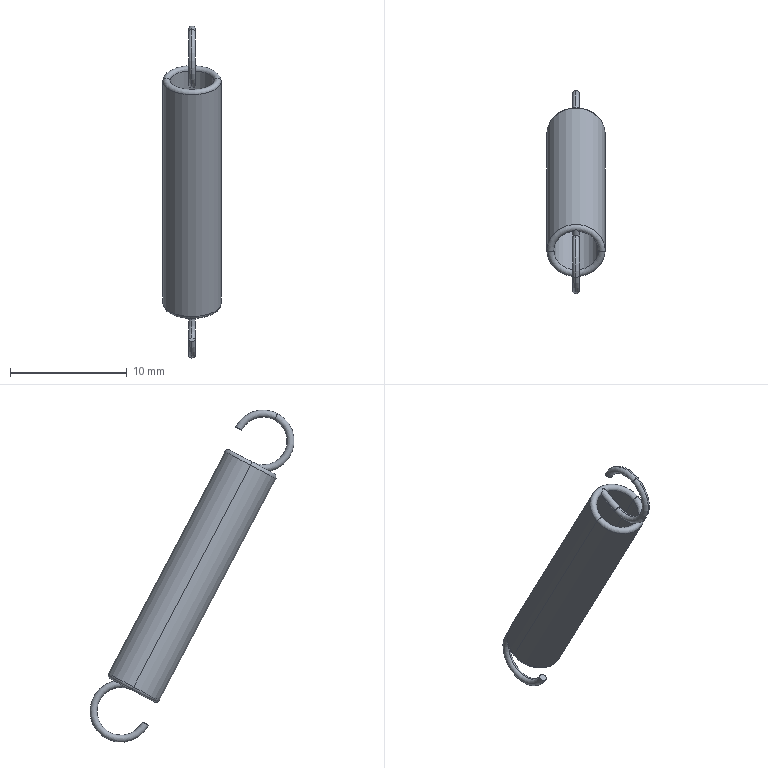Component | SolidWorks | LiftingPlateAssembly-1_AWS5_30-2 | 1 solid | 20 faces | box 5 x 17.5 x 28.48 mm | volume 190 mm3 | torus 10 | cylinder 8 | plane 2 | commonest cylinder face diameters 0.6 x4 5 x2 3.8 x2
build123d program:
from build123d import *

# Parameters (mm, degrees)
SKETCH2_W      = 0.3
SKETCH2_H      = 2.2
SKETCH3_R      = 0.3
REVOLVE3_ANGLE = 271
SKETCH4_W      = 0.3
SKETCH4_H      = 2.2
SKETCH5_R      = 0.3
REVOLVE5_ANGLE = 271


with BuildPart() as part:
    # Sketch1 → Revolve1 (revolve)
    with BuildSketch(Plane.XY, mode=Mode.PRIVATE) as revolve1_sk:
        with BuildLine():
            Line((4.25, 2.5), (25.75, 2.5))
            ThreePointArc((25.75, 2.5), (26.05, 2.2), (25.75, 1.9))
            Line((25.75, 1.9), (4.25, 1.9))
            ThreePointArc((4.25, 1.9), (3.95, 2.2), (4.25, 2.5))
        make_face()
    revolve(revolve1_sk.sketch.rotate(Axis((26.2, 0, 0), (-1, 0, 0)), 270), axis=Axis((26.2, 0, 0), (-1, 0, 0)))

    # Sketch2 → Revolve2 (revolve)
    with BuildSketch(Plane.XY, mode=Mode.PRIVATE) as revolve2_sk:
        with Locations((25.9, 1.1)):
            Rectangle(SKETCH2_W, SKETCH2_H)
    revolve(revolve2_sk.sketch.rotate(Axis((25.75, 0, 0), (0, 1, 0)), 270), axis=Axis((25.75, 0, 0), (0, 1, 0)))

    # Sketch3 → Revolve3 (revolve)
    with BuildSketch(Plane(origin=(0, 0, 0), x_dir=(1, 0, 0), z_dir=(0, 1, 0))):
        with Locations(Location((25.75, 0, 0), (0, 0, 270))):
            Circle(SKETCH3_R)
    revolve(axis=Axis((28.1, 0, -2.5), (0, 0, 1)), revolution_arc=REVOLVE3_ANGLE)

    # Sketch4 → Revolve4 (revolve)
    with BuildSketch(Plane.XY, mode=Mode.PRIVATE) as revolve4_sk:
        with Locations((4.4, -1.1)):
            Rectangle(SKETCH4_W, SKETCH4_H)
    revolve(revolve4_sk.sketch.rotate(Axis((4.25, 0, 0), (0, -1, 0)), 90), axis=Axis((4.25, 0, 0), (0, -1, 0)))

    # Sketch5 → Revolve5 (revolve)
    with BuildSketch(Plane(origin=(0, 0, 0), x_dir=(1, 0, 0), z_dir=(0, 1, 0))):
        with Locations(Location((4.25, 0, 0), (0, 0, 270))):
            Circle(SKETCH5_R)
    revolve(axis=Axis((1.9, 0, 2.5), (0, 0, 1)), revolution_arc=REVOLVE5_ANGLE)


solid = part.part

# Placed as in the assembly
solid = solid.moved(Location((-282.5, -21.911, -69.866), (27.761, -90, 0)))
STEP:
#1=CARTESIAN_POINT('',(-11.122,-1.427,-1.679));
#2=VERTEX_POINT('',#1);
#3=CARTESIAN_POINT('',(-11.122,-1.416,-1.7));
#4=VERTEX_POINT('',#3);
#5=CARTESIAN_POINT('',(-11.122,-1.421,-1.69));
#6=DIRECTION('',(-0.,0.8849,0.4658));
#7=DIRECTION('',(0.,-0.4658,0.8849));
#8=AXIS2_PLACEMENT_3D('',#5,#6,#7);
#9=CIRCLE('',#8,0.01181);
#10=EDGE_CURVE('',#2,#4,#9,.T.);
#11=ORIENTED_EDGE('',*,*,#10,.F.);
#12=CARTESIAN_POINT('',(-11.122,-1.329,-1.864));
#13=VERTEX_POINT('',#12);
#14=CARTESIAN_POINT('',(-11.122,-1.378,-1.772));
#15=DIRECTION('',(1.,0.,-0.));
#16=DIRECTION('',(0.,1.,0.));
#17=AXIS2_PLACEMENT_3D('',#14,#15,#16);
#18=CIRCLE('',#17,0.1043);
#19=EDGE_CURVE('',#2,#13,#18,.T.);
#20=ORIENTED_EDGE('',*,*,#19,.T.);
#21=CARTESIAN_POINT('',(-11.11,-1.335,-1.854));
#22=VERTEX_POINT('',#21);
#23=CARTESIAN_POINT('',(-11.122,-1.335,-1.854));
#24=DIRECTION('',(0.,-0.8849,-0.4658));
#25=DIRECTION('',(-1.,0.,0.));
#26=AXIS2_PLACEMENT_3D('',#23,#24,#25);
#27=CIRCLE('',#26,0.01181);
#28=EDGE_CURVE('',#13,#22,#27,.T.);
#29=ORIENTED_EDGE('',*,*,#28,.T.);
#30=CARTESIAN_POINT('',(-11.122,-1.34,-1.843));
#31=VERTEX_POINT('',#30);
#32=CARTESIAN_POINT('',(-11.122,-1.335,-1.854));
#33=DIRECTION('',(0.,-0.8849,-0.4658));
#34=DIRECTION('',(-1.,0.,0.));
#35=AXIS2_PLACEMENT_3D('',#32,#33,#34);
#36=CIRCLE('',#35,0.01181);
#37=EDGE_CURVE('',#22,#31,#36,.T.);
#38=ORIENTED_EDGE('',*,*,#37,.T.);
#39=CARTESIAN_POINT('',(-11.122,-1.378,-1.772));
#40=DIRECTION('',(1.,0.,-0.));
#41=DIRECTION('',(0.,1.,0.));
#42=AXIS2_PLACEMENT_3D('',#39,#40,#41);
#43=CIRCLE('',#42,0.08071);
#44=EDGE_CURVE('',#4,#31,#43,.T.);
#45=ORIENTED_EDGE('',*,*,#44,.F.);
#46=EDGE_LOOP('',(#11,#20,#29,#38,#45));
#47=FACE_OUTER_BOUND('',#46,.T.);
#48=CARTESIAN_POINT('',(-11.122,-1.378,-1.772));
#49=DIRECTION('',(1.,0.,-0.));
#50=DIRECTION('',(0.,-0.4658,0.8849));
#51=AXIS2_PLACEMENT_3D('',#48,#49,#50);
#52=TOROIDAL_SURFACE('',#51,0.09252,0.01181);
#53=ADVANCED_FACE('',(#47),#52,.T.);
#54=CARTESIAN_POINT('',(-11.122,-0.9696,-2.721));
#55=VERTEX_POINT('',#54);
#56=CARTESIAN_POINT('',(-11.122,-0.9907,-2.731));
#57=VERTEX_POINT('',#56);
#58=CARTESIAN_POINT('',(-11.122,-0.9801,-2.726));
#59=DIRECTION('',(-0.,0.4503,-0.8929));
#60=DIRECTION('',(-1.,0.,0.));
#61=AXIS2_PLACEMENT_3D('',#58,#59,#60);
#62=CIRCLE('',#61,0.01181);
#63=EDGE_CURVE('',#55,#57,#62,.T.);
#64=ORIENTED_EDGE('',*,*,#63,.T.);
#65=CARTESIAN_POINT('',(-11.122,-0.9461,-2.592));
#66=VERTEX_POINT('',#65);
#67=CARTESIAN_POINT('',(-11.122,-0.8975,-2.684));
#68=DIRECTION('',(1.,0.,-0.));
#69=DIRECTION('',(0.,1.,0.));
#70=AXIS2_PLACEMENT_3D('',#67,#68,#69);
#71=CIRCLE('',#70,0.1043);
#72=EDGE_CURVE('',#57,#66,#71,.T.);
#73=ORIENTED_EDGE('',*,*,#72,.T.);
#74=CARTESIAN_POINT('',(-11.11,-0.9406,-2.603));
#75=VERTEX_POINT('',#74);
#76=CARTESIAN_POINT('',(-11.122,-0.9406,-2.603));
#77=DIRECTION('',(0.,-0.8849,-0.4658));
#78=DIRECTION('',(-1.,0.,0.));
#79=AXIS2_PLACEMENT_3D('',#76,#77,#78);
#80=CIRCLE('',#79,0.01181);
#81=EDGE_CURVE('',#75,#66,#80,.T.);
#82=ORIENTED_EDGE('',*,*,#81,.F.);
#83=CARTESIAN_POINT('',(-11.122,-0.9351,-2.613));
#84=VERTEX_POINT('',#83);
#85=CARTESIAN_POINT('',(-11.122,-0.9406,-2.603));
#86=DIRECTION('',(0.,-0.8849,-0.4658));
#87=DIRECTION('',(-1.,0.,0.));
#88=AXIS2_PLACEMENT_3D('',#85,#86,#87);
#89=CIRCLE('',#88,0.01181);
#90=EDGE_CURVE('',#84,#75,#89,.T.);
#91=ORIENTED_EDGE('',*,*,#90,.F.);
#92=CARTESIAN_POINT('',(-11.122,-0.8975,-2.684));
#93=DIRECTION('',(1.,0.,-0.));
#94=DIRECTION('',(0.,1.,0.));
#95=AXIS2_PLACEMENT_3D('',#92,#93,#94);
#96=CIRCLE('',#95,0.08071);
#97=EDGE_CURVE('',#55,#84,#96,.T.);
#98=ORIENTED_EDGE('',*,*,#97,.F.);
#99=EDGE_LOOP('',(#64,#73,#82,#91,#98));
#100=FACE_OUTER_BOUND('',#99,.T.);
#101=CARTESIAN_POINT('',(-11.122,-0.8975,-2.684));
#102=DIRECTION('',(1.,0.,-0.));
#103=DIRECTION('',(0.,-0.4658,0.8849));
#104=AXIS2_PLACEMENT_3D('',#101,#102,#103);
#105=TOROIDAL_SURFACE('',#104,0.09252,0.01181);
#106=ADVANCED_FACE('',(#100),#105,.T.);
#107=CARTESIAN_POINT('',(-11.122,-1.285,-1.725));
#108=VERTEX_POINT('',#107);
#109=CARTESIAN_POINT('',(-11.122,-1.306,-1.735));
#110=VERTEX_POINT('',#109);
#111=CARTESIAN_POINT('',(-11.122,-1.295,-1.73));
#112=DIRECTION('',(-0.,0.4503,-0.8929));
#113=DIRECTION('',(-1.,0.,0.));
#114=AXIS2_PLACEMENT_3D('',#111,#112,#113);
#115=CIRCLE('',#114,0.01181);
#116=EDGE_CURVE('',#108,#110,#115,.T.);
#117=ORIENTED_EDGE('',*,*,#116,.F.);
#118=CARTESIAN_POINT('',(-11.122,-1.378,-1.772));
#119=DIRECTION('',(1.,0.,-0.));
#120=DIRECTION('',(0.,1.,0.));
#121=AXIS2_PLACEMENT_3D('',#118,#119,#120);
#122=CIRCLE('',#121,0.1043);
#123=EDGE_CURVE('',#108,#2,#122,.T.);
#124=ORIENTED_EDGE('',*,*,#123,.T.);
#125=ORIENTED_EDGE('',*,*,#10,.T.);
#126=CARTESIAN_POINT('',(-11.122,-1.378,-1.772));
#127=DIRECTION('',(1.,0.,-0.));
#128=DIRECTION('',(0.,1.,0.));
#129=AXIS2_PLACEMENT_3D('',#126,#127,#128);
#130=CIRCLE('',#129,0.08071);
#131=EDGE_CURVE('',#110,#4,#130,.T.);
#132=ORIENTED_EDGE('',*,*,#131,.F.);
#133=EDGE_LOOP('',(#117,#124,#125,#132));
#134=FACE_OUTER_BOUND('',#133,.T.);
#135=CARTESIAN_POINT('',(-11.122,-1.378,-1.772));
#136=DIRECTION('',(1.,0.,-0.));
#137=DIRECTION('',(0.,-0.4658,0.8849));
#138=AXIS2_PLACEMENT_3D('',#135,#136,#137);
#139=TOROIDAL_SURFACE('',#138,0.09252,0.01181);
#140=ADVANCED_FACE('',(#134),#139,.T.);
#141=ORIENTED_EDGE('',*,*,#123,.F.);
#142=CARTESIAN_POINT('',(-11.122,-1.295,-1.73));
#143=DIRECTION('',(-0.,0.4503,-0.8929));
#144=DIRECTION('',(-1.,0.,0.));
#145=AXIS2_PLACEMENT_3D('',#142,#143,#144);
#146=CIRCLE('',#145,0.01181);
#147=EDGE_CURVE('',#110,#108,#146,.T.);
#148=ORIENTED_EDGE('',*,*,#147,.F.);
#149=ORIENTED_EDGE('',*,*,#131,.T.);
#150=CARTESIAN_POINT('',(-11.122,-1.421,-1.69));
#151=DIRECTION('',(-0.,0.8849,0.4658));
#152=DIRECTION('',(0.,-0.4658,0.8849));
#153=AXIS2_PLACEMENT_3D('',#150,#151,#152);
#154=CIRCLE('',#153,0.01181);
#155=EDGE_CURVE('',#4,#2,#154,.T.);
#156=ORIENTED_EDGE('',*,*,#155,.T.);
#157=EDGE_LOOP('',(#141,#148,#149,#156));
#158=FACE_OUTER_BOUND('',#157,.T.);
#159=CARTESIAN_POINT('',(-11.122,-1.378,-1.772));
#160=DIRECTION('',(1.,0.,-0.));
#161=DIRECTION('',(0.,-0.4658,0.8849));
#162=AXIS2_PLACEMENT_3D('',#159,#160,#161);
#163=TOROIDAL_SURFACE('',#162,0.09252,0.01181);
#164=ADVANCED_FACE('',(#158),#163,.T.);
#165=CARTESIAN_POINT('',(-11.134,-1.269,-1.819));
#166=VERTEX_POINT('',#165);
#167=CARTESIAN_POINT('',(-11.11,-1.269,-1.819));
#168=VERTEX_POINT('',#167);
#169=CARTESIAN_POINT('',(-11.134,-1.269,-1.819));
#170=CARTESIAN_POINT('',(-11.134,-1.268,-1.822));
#171=CARTESIAN_POINT('',(-11.133,-1.266,-1.824));
#172=CARTESIAN_POINT('',(-11.128,-1.264,-1.828));
#173=CARTESIAN_POINT('',(-11.125,-1.263,-1.829));
#174=CARTESIAN_POINT('',(-11.119,-1.263,-1.829));
#175=CARTESIAN_POINT('',(-11.116,-1.264,-1.828));
#176=CARTESIAN_POINT('',(-11.111,-1.266,-1.824));
#177=CARTESIAN_POINT('',(-11.11,-1.268,-1.822));
#178=CARTESIAN_POINT('',(-11.11,-1.269,-1.819));
#179=B_SPLINE_CURVE_WITH_KNOTS('',3,(#169,#170,#171,#172,#173,#174,#175,#176,#177,#178),.UNSPECIFIED.,.F.,.F.,(4,2,2,2,4),(0.,0.0002349,0.0004697,0.0007046,0.0009394),.UNSPECIFIED.);
#180=EDGE_CURVE('',#166,#168,#179,.T.);
#181=ORIENTED_EDGE('',*,*,#180,.T.);
#182=CARTESIAN_POINT('',(-11.11,-1.335,-1.854));
#183=DIRECTION('',(0.,-0.8849,-0.4658));
#184=VECTOR('',#183,39.37);
#185=LINE('',#182,#184);
#186=EDGE_CURVE('',#168,#22,#185,.T.);
#187=ORIENTED_EDGE('',*,*,#186,.T.);
#188=ORIENTED_EDGE('',*,*,#28,.F.);
#189=CARTESIAN_POINT('',(-11.134,-1.335,-1.854));
#190=VERTEX_POINT('',#189);
#191=CARTESIAN_POINT('',(-11.122,-1.335,-1.854));
#192=DIRECTION('',(0.,-0.8849,-0.4658));
#193=DIRECTION('',(-1.,0.,0.));
#194=AXIS2_PLACEMENT_3D('',#191,#192,#193);
#195=CIRCLE('',#194,0.01181);
#196=EDGE_CURVE('',#190,#13,#195,.T.);
#197=ORIENTED_EDGE('',*,*,#196,.F.);
#198=CARTESIAN_POINT('',(-11.134,-1.335,-1.854));
#199=DIRECTION('',(0.,-0.8849,-0.4658));
#200=VECTOR('',#199,39.37);
#201=LINE('',#198,#200);
#202=EDGE_CURVE('',#166,#190,#201,.T.);
#203=ORIENTED_EDGE('',*,*,#202,.F.);
#204=EDGE_LOOP('',(#181,#187,#188,#197,#203));
#205=FACE_OUTER_BOUND('',#204,.T.);
#206=CARTESIAN_POINT('',(-11.122,-1.335,-1.854));
#207=DIRECTION('',(0.,-0.8849,-0.4658));
#208=DIRECTION('',(-1.,0.,0.));
#209=AXIS2_PLACEMENT_3D('',#206,#207,#208);
#210=CYLINDRICAL_SURFACE('',#209,0.01181);
#211=ADVANCED_FACE('',(#205),#210,.T.);
#212=CARTESIAN_POINT('',(-11.134,-0.9406,-2.603));
#213=VERTEX_POINT('',#212);
#214=CARTESIAN_POINT('',(-11.122,-0.9406,-2.603));
#215=DIRECTION('',(0.,-0.8849,-0.4658));
#216=DIRECTION('',(-1.,0.,0.));
#217=AXIS2_PLACEMENT_3D('',#214,#215,#216);
#218=CIRCLE('',#217,0.01181);
#219=EDGE_CURVE('',#213,#84,#218,.T.);
#220=ORIENTED_EDGE('',*,*,#219,.T.);
#221=ORIENTED_EDGE('',*,*,#90,.T.);
#222=CARTESIAN_POINT('',(-11.11,-1.006,-2.637));
#223=VERTEX_POINT('',#222);
#224=CARTESIAN_POINT('',(-11.11,-0.9406,-2.603));
#225=DIRECTION('',(0.,-0.8849,-0.4658));
#226=VECTOR('',#225,39.37);
#227=LINE('',#224,#226);
#228=EDGE_CURVE('',#75,#223,#227,.T.);
#229=ORIENTED_EDGE('',*,*,#228,.T.);
#230=CARTESIAN_POINT('',(-11.122,-1.012,-2.653));
#231=VERTEX_POINT('',#230);
#232=CARTESIAN_POINT('',(-11.11,-1.006,-2.637));
#233=CARTESIAN_POINT('',(-11.11,-1.005,-2.639));
#234=CARTESIAN_POINT('',(-11.111,-1.005,-2.641));
#235=CARTESIAN_POINT('',(-11.112,-1.005,-2.644));
#236=CARTESIAN_POINT('',(-11.113,-1.005,-2.646));
#237=CARTESIAN_POINT('',(-11.117,-1.007,-2.65));
#238=CARTESIAN_POINT('',(-11.119,-1.009,-2.652));
#239=CARTESIAN_POINT('',(-11.122,-1.012,-2.653));
#240=B_SPLINE_CURVE_WITH_KNOTS('',3,(#232,#233,#234,#235,#236,#237,#238,#239),.UNSPECIFIED.,.F.,.F.,(4,2,2,4),(0.0000002,0.0001461,0.000292,0.0005837),.UNSPECIFIED.);
#241=EDGE_CURVE('',#223,#231,#240,.T.);
#242=ORIENTED_EDGE('',*,*,#241,.T.);
#243=CARTESIAN_POINT('',(-11.134,-1.006,-2.637));
#244=VERTEX_POINT('',#243);
#245=CARTESIAN_POINT('',(-11.122,-1.012,-2.653));
#246=CARTESIAN_POINT('',(-11.125,-1.009,-2.652));
#247=CARTESIAN_POINT('',(-11.127,-1.007,-2.65));
#248=CARTESIAN_POINT('',(-11.131,-1.005,-2.646));
#249=CARTESIAN_POINT('',(-11.132,-1.005,-2.644));
#250=CARTESIAN_POINT('',(-11.133,-1.005,-2.641));
#251=CARTESIAN_POINT('',(-11.134,-1.005,-2.639));
#252=CARTESIAN_POINT('',(-11.134,-1.006,-2.637));
#253=B_SPLINE_CURVE_WITH_KNOTS('',3,(#245,#246,#247,#248,#249,#250,#251,#252),.UNSPECIFIED.,.F.,.F.,(4,2,2,4),(-0.00000346,0.0002869,0.0004321,0.0005772),.UNSPECIFIED.);
#254=EDGE_CURVE('',#231,#244,#253,.T.);
#255=ORIENTED_EDGE('',*,*,#254,.T.);
#256=CARTESIAN_POINT('',(-11.134,-0.9406,-2.603));
#257=DIRECTION('',(0.,-0.8849,-0.4658));
#258=VECTOR('',#257,39.37);
#259=LINE('',#256,#258);
#260=EDGE_CURVE('',#213,#244,#259,.T.);
#261=ORIENTED_EDGE('',*,*,#260,.F.);
#262=EDGE_LOOP('',(#220,#221,#229,#242,#255,#261));
#263=FACE_OUTER_BOUND('',#262,.T.);
#264=CARTESIAN_POINT('',(-11.122,-0.9406,-2.603));
#265=DIRECTION('',(0.,-0.8849,-0.4658));
#266=DIRECTION('',(-1.,0.,0.));
#267=AXIS2_PLACEMENT_3D('',#264,#265,#266);
#268=CYLINDRICAL_SURFACE('',#267,0.01181);
#269=ADVANCED_FACE('',(#263),#268,.T.);
#270=CARTESIAN_POINT('',(-11.22,-0.9406,-2.603));
#271=VERTEX_POINT('',#270);
#272=CARTESIAN_POINT('',(-11.024,-0.9406,-2.603));
#273=VERTEX_POINT('',#272);
#274=CARTESIAN_POINT('',(-11.122,-0.9406,-2.603));
#275=DIRECTION('',(0.,-0.4658,0.8849));
#276=DIRECTION('',(-1.,0.,0.));
#277=AXIS2_PLACEMENT_3D('',#274,#275,#276);
#278=CIRCLE('',#277,0.09843);
#279=EDGE_CURVE('',#271,#273,#278,.T.);
#280=ORIENTED_EDGE('',*,*,#279,.T.);
#281=CARTESIAN_POINT('',(-11.024,-1.335,-1.854));
#282=VERTEX_POINT('',#281);
#283=CARTESIAN_POINT('',(-11.024,-0.9323,-2.618));
#284=DIRECTION('',(0.,-0.4658,0.8849));
#285=VECTOR('',#284,39.37);
#286=LINE('',#283,#285);
#287=EDGE_CURVE('',#273,#282,#286,.T.);
#288=ORIENTED_EDGE('',*,*,#287,.T.);
#289=CARTESIAN_POINT('',(-11.22,-1.335,-1.854));
#290=VERTEX_POINT('',#289);
#291=CARTESIAN_POINT('',(-11.122,-1.335,-1.854));
#292=DIRECTION('',(0.,-0.4658,0.8849));
#293=DIRECTION('',(-1.,0.,0.));
#294=AXIS2_PLACEMENT_3D('',#291,#292,#293);
#295=CIRCLE('',#294,0.09843);
#296=EDGE_CURVE('',#290,#282,#295,.T.);
#297=ORIENTED_EDGE('',*,*,#296,.F.);
#298=CARTESIAN_POINT('',(-11.22,-0.9323,-2.618));
#299=DIRECTION('',(0.,-0.4658,0.8849));
#300=VECTOR('',#299,39.37);
#301=LINE('',#298,#300);
#302=EDGE_CURVE('',#271,#290,#301,.T.);
#303=ORIENTED_EDGE('',*,*,#302,.F.);
#304=EDGE_LOOP('',(#280,#288,#297,#303));
#305=FACE_OUTER_BOUND('',#304,.T.);
#306=CARTESIAN_POINT('',(-11.122,-0.9323,-2.618));
#307=DIRECTION('',(0.,-0.4658,0.8849));
#308=DIRECTION('',(-1.,0.,0.));
#309=AXIS2_PLACEMENT_3D('',#306,#307,#308);
#310=CYLINDRICAL_SURFACE('',#309,0.09843);
#311=ADVANCED_FACE('',(#305),#310,.T.);
#312=CARTESIAN_POINT('',(-11.047,-0.9406,-2.603));
#313=VERTEX_POINT('',#312);
#314=CARTESIAN_POINT('',(-11.122,-0.9406,-2.603));
#315=DIRECTION('',(0.,-0.4658,0.8849));
#316=DIRECTION('',(-1.,0.,0.));
#317=AXIS2_PLACEMENT_3D('',#314,#315,#316);
#318=CIRCLE('',#317,0.0748);
#319=EDGE_CURVE('',#223,#313,#318,.T.);
#320=ORIENTED_EDGE('',*,*,#319,.T.);
#321=CARTESIAN_POINT('',(-11.035,-0.9406,-2.603));
#322=DIRECTION('',(0.,-0.8849,-0.4658));
#323=DIRECTION('',(0.,0.4658,-0.8849));
#324=AXIS2_PLACEMENT_3D('',#321,#322,#323);
#325=CIRCLE('',#324,0.01181);
#326=EDGE_CURVE('',#313,#273,#325,.T.);
#327=ORIENTED_EDGE('',*,*,#326,.T.);
#328=ORIENTED_EDGE('',*,*,#279,.F.);
#329=CARTESIAN_POINT('',(-11.197,-0.9406,-2.603));
#330=VERTEX_POINT('',#329);
#331=CARTESIAN_POINT('',(-11.209,-0.9406,-2.603));
#332=DIRECTION('',(-0.,0.8849,0.4658));
#333=DIRECTION('',(0.,-0.4658,0.8849));
#334=AXIS2_PLACEMENT_3D('',#331,#332,#333);
#335=CIRCLE('',#334,0.01181);
#336=EDGE_CURVE('',#330,#271,#335,.T.);
#337=ORIENTED_EDGE('',*,*,#336,.F.);
#338=CARTESIAN_POINT('',(-11.122,-0.9406,-2.603));
#339=DIRECTION('',(0.,-0.4658,0.8849));
#340=DIRECTION('',(-1.,0.,0.));
#341=AXIS2_PLACEMENT_3D('',#338,#339,#340);
#342=CIRCLE('',#341,0.0748);
#343=EDGE_CURVE('',#330,#244,#342,.T.);
#344=ORIENTED_EDGE('',*,*,#343,.T.);
#345=ORIENTED_EDGE('',*,*,#254,.F.);
#346=ORIENTED_EDGE('',*,*,#241,.F.);
#347=EDGE_LOOP('',(#320,#327,#328,#337,#344,#345,#346));
#348=FACE_OUTER_BOUND('',#347,.T.);
#349=CARTESIAN_POINT('',(-11.122,-0.9406,-2.603));
#350=DIRECTION('',(0.,-0.4658,0.8849));
#351=DIRECTION('',(-1.,-0.,0.));
#352=AXIS2_PLACEMENT_3D('',#349,#350,#351);
#353=TOROIDAL_SURFACE('',#352,0.08661,0.01181);
#354=ADVANCED_FACE('',(#348),#353,.T.);
#355=ORIENTED_EDGE('',*,*,#296,.T.);
#356=CARTESIAN_POINT('',(-11.047,-1.335,-1.854));
#357=VERTEX_POINT('',#356);
#358=CARTESIAN_POINT('',(-11.035,-1.335,-1.854));
#359=DIRECTION('',(0.,-0.8849,-0.4658));
#360=DIRECTION('',(0.,0.4658,-0.8849));
#361=AXIS2_PLACEMENT_3D('',#358,#359,#360);
#362=CIRCLE('',#361,0.01181);
#363=EDGE_CURVE('',#282,#357,#362,.T.);
#364=ORIENTED_EDGE('',*,*,#363,.T.);
#365=CARTESIAN_POINT('',(-11.197,-1.335,-1.854));
#366=VERTEX_POINT('',#365);
#367=CARTESIAN_POINT('',(-11.122,-1.335,-1.854));
#368=DIRECTION('',(0.,-0.4658,0.8849));
#369=DIRECTION('',(-1.,0.,0.));
#370=AXIS2_PLACEMENT_3D('',#367,#368,#369);
#371=CIRCLE('',#370,0.0748);
#372=EDGE_CURVE('',#366,#357,#371,.T.);
#373=ORIENTED_EDGE('',*,*,#372,.F.);
#374=CARTESIAN_POINT('',(-11.209,-1.335,-1.854));
#375=DIRECTION('',(-0.,0.8849,0.4658));
#376=DIRECTION('',(0.,-0.4658,0.8849));
#377=AXIS2_PLACEMENT_3D('',#374,#375,#376);
#378=CIRCLE('',#377,0.01181);
#379=EDGE_CURVE('',#290,#366,#378,.T.);
#380=ORIENTED_EDGE('',*,*,#379,.F.);
#381=EDGE_LOOP('',(#355,#364,#373,#380));
#382=FACE_OUTER_BOUND('',#381,.T.);
#383=CARTESIAN_POINT('',(-11.122,-1.335,-1.854));
#384=DIRECTION('',(0.,-0.4658,0.8849));
#385=DIRECTION('',(-1.,-0.,0.));
#386=AXIS2_PLACEMENT_3D('',#383,#384,#385);
#387=TOROIDAL_SURFACE('',#386,0.08661,0.01181);
#388=ADVANCED_FACE('',(#382),#387,.T.);
#389=CARTESIAN_POINT('',(-11.122,-0.9406,-2.603));
#390=DIRECTION('',(0.,-0.4658,0.8849));
#391=DIRECTION('',(-1.,0.,0.));
#392=AXIS2_PLACEMENT_3D('',#389,#390,#391);
#393=CIRCLE('',#392,0.0748);
#394=EDGE_CURVE('',#313,#330,#393,.T.);
#395=ORIENTED_EDGE('',*,*,#394,.F.);
#396=CARTESIAN_POINT('',(-11.047,-0.9323,-2.618));
#397=DIRECTION('',(0.,-0.4658,0.8849));
#398=VECTOR('',#397,39.37);
#399=LINE('',#396,#398);
#400=EDGE_CURVE('',#313,#357,#399,.T.);
#401=ORIENTED_EDGE('',*,*,#400,.T.);
#402=CARTESIAN_POINT('',(-11.122,-1.335,-1.854));
#403=DIRECTION('',(0.,-0.4658,0.8849));
#404=DIRECTION('',(-1.,0.,0.));
#405=AXIS2_PLACEMENT_3D('',#402,#403,#404);
#406=CIRCLE('',#405,0.0748);
#407=EDGE_CURVE('',#357,#168,#406,.T.);
#408=ORIENTED_EDGE('',*,*,#407,.T.);
#409=ORIENTED_EDGE('',*,*,#180,.F.);
#410=CARTESIAN_POINT('',(-11.122,-1.335,-1.854));
#411=DIRECTION('',(0.,-0.4658,0.8849));
#412=DIRECTION('',(-1.,0.,0.));
#413=AXIS2_PLACEMENT_3D('',#410,#411,#412);
#414=CIRCLE('',#413,0.0748);
#415=EDGE_CURVE('',#166,#366,#414,.T.);
#416=ORIENTED_EDGE('',*,*,#415,.T.);
#417=CARTESIAN_POINT('',(-11.197,-0.9323,-2.618));
#418=DIRECTION('',(0.,-0.4658,0.8849));
#419=VECTOR('',#418,39.37);
#420=LINE('',#417,#419);
#421=EDGE_CURVE('',#330,#366,#420,.T.);
#422=ORIENTED_EDGE('',*,*,#421,.F.);
#423=EDGE_LOOP('',(#395,#401,#408,#409,#416,#422));
#424=FACE_OUTER_BOUND('',#423,.T.);
#425=CARTESIAN_POINT('',(-11.122,-0.9323,-2.618));
#426=DIRECTION('',(0.,-0.4658,0.8849));
#427=DIRECTION('',(-1.,0.,0.));
#428=AXIS2_PLACEMENT_3D('',#425,#426,#427);
#429=CYLINDRICAL_SURFACE('',#428,0.0748);
#430=ADVANCED_FACE('',(#424),#429,.F.);
#431=ORIENTED_EDGE('',*,*,#400,.F.);
#432=ORIENTED_EDGE('',*,*,#319,.F.);
#433=CARTESIAN_POINT('',(-11.134,-1.006,-2.637));
#434=CARTESIAN_POINT('',(-11.134,-1.007,-2.634));
#435=CARTESIAN_POINT('',(-11.133,-1.009,-2.632));
#436=CARTESIAN_POINT('',(-11.128,-1.011,-2.628));
#437=CARTESIAN_POINT('',(-11.125,-1.012,-2.627));
#438=CARTESIAN_POINT('',(-11.119,-1.012,-2.627));
#439=CARTESIAN_POINT('',(-11.116,-1.012,-2.628));
#440=CARTESIAN_POINT('',(-11.111,-1.009,-2.632));
#441=CARTESIAN_POINT('',(-11.11,-1.007,-2.634));
#442=CARTESIAN_POINT('',(-11.11,-1.006,-2.637));
#443=B_SPLINE_CURVE_WITH_KNOTS('',3,(#433,#434,#435,#436,#437,#438,#439,#440,#441,#442),.UNSPECIFIED.,.F.,.F.,(4,2,2,2,4),(0.,0.0002349,0.0004697,0.0007046,0.0009394),.UNSPECIFIED.);
#444=EDGE_CURVE('',#244,#223,#443,.T.);
#445=ORIENTED_EDGE('',*,*,#444,.F.);
#446=ORIENTED_EDGE('',*,*,#343,.F.);
#447=ORIENTED_EDGE('',*,*,#421,.T.);
#448=ORIENTED_EDGE('',*,*,#372,.T.);
#449=EDGE_LOOP('',(#431,#432,#445,#446,#447,#448));
#450=FACE_OUTER_BOUND('',#449,.T.);
#451=CARTESIAN_POINT('',(-11.122,-0.9323,-2.618));
#452=DIRECTION('',(0.,-0.4658,0.8849));
#453=DIRECTION('',(-1.,0.,0.));
#454=AXIS2_PLACEMENT_3D('',#451,#452,#453);
#455=CYLINDRICAL_SURFACE('',#454,0.0748);
#456=ADVANCED_FACE('',(#450),#455,.F.);
#457=ORIENTED_EDGE('',*,*,#363,.F.);
#458=CARTESIAN_POINT('',(-11.122,-1.335,-1.854));
#459=DIRECTION('',(0.,-0.4658,0.8849));
#460=DIRECTION('',(-1.,0.,0.));
#461=AXIS2_PLACEMENT_3D('',#458,#459,#460);
#462=CIRCLE('',#461,0.09843);
#463=EDGE_CURVE('',#282,#290,#462,.T.);
#464=ORIENTED_EDGE('',*,*,#463,.T.);
#465=ORIENTED_EDGE('',*,*,#379,.T.);
#466=ORIENTED_EDGE('',*,*,#415,.F.);
#467=CARTESIAN_POINT('',(-11.122,-1.264,-1.803));
#468=VERTEX_POINT('',#467);
#469=CARTESIAN_POINT('',(-11.122,-1.264,-1.803));
#470=CARTESIAN_POINT('',(-11.125,-1.266,-1.804));
#471=CARTESIAN_POINT('',(-11.127,-1.268,-1.806));
#472=CARTESIAN_POINT('',(-11.131,-1.27,-1.81));
#473=CARTESIAN_POINT('',(-11.132,-1.271,-1.812));
#474=CARTESIAN_POINT('',(-11.133,-1.271,-1.815));
#475=CARTESIAN_POINT('',(-11.134,-1.27,-1.817));
#476=CARTESIAN_POINT('',(-11.134,-1.269,-1.819));
#477=B_SPLINE_CURVE_WITH_KNOTS('',3,(#469,#470,#471,#472,#473,#474,#475,#476),.UNSPECIFIED.,.F.,.F.,(4,2,2,4),(-0.00000346,0.0002869,0.0004321,0.0005772),.UNSPECIFIED.);
#478=EDGE_CURVE('',#468,#166,#477,.T.);
#479=ORIENTED_EDGE('',*,*,#478,.F.);
#480=CARTESIAN_POINT('',(-11.11,-1.269,-1.819));
#481=CARTESIAN_POINT('',(-11.11,-1.27,-1.817));
#482=CARTESIAN_POINT('',(-11.111,-1.271,-1.815));
#483=CARTESIAN_POINT('',(-11.112,-1.271,-1.812));
#484=CARTESIAN_POINT('',(-11.113,-1.27,-1.81));
#485=CARTESIAN_POINT('',(-11.117,-1.268,-1.806));
#486=CARTESIAN_POINT('',(-11.119,-1.266,-1.804));
#487=CARTESIAN_POINT('',(-11.122,-1.264,-1.803));
#488=B_SPLINE_CURVE_WITH_KNOTS('',3,(#480,#481,#482,#483,#484,#485,#486,#487),.UNSPECIFIED.,.F.,.F.,(4,2,2,4),(0.0000002,0.0001461,0.000292,0.0005837),.UNSPECIFIED.);
#489=EDGE_CURVE('',#168,#468,#488,.T.);
#490=ORIENTED_EDGE('',*,*,#489,.F.);
#491=ORIENTED_EDGE('',*,*,#407,.F.);
#492=EDGE_LOOP('',(#457,#464,#465,#466,#479,#490,#491));
#493=FACE_OUTER_BOUND('',#492,.T.);
#494=CARTESIAN_POINT('',(-11.122,-1.335,-1.854));
#495=DIRECTION('',(0.,-0.4658,0.8849));
#496=DIRECTION('',(-1.,-0.,0.));
#497=AXIS2_PLACEMENT_3D('',#494,#495,#496);
#498=TOROIDAL_SURFACE('',#497,0.08661,0.01181);
#499=ADVANCED_FACE('',(#493),#498,.T.);
#500=ORIENTED_EDGE('',*,*,#326,.F.);
#501=ORIENTED_EDGE('',*,*,#394,.T.);
#502=ORIENTED_EDGE('',*,*,#336,.T.);
#503=CARTESIAN_POINT('',(-11.122,-0.9406,-2.603));
#504=DIRECTION('',(0.,-0.4658,0.8849));
#505=DIRECTION('',(-1.,0.,0.));
#506=AXIS2_PLACEMENT_3D('',#503,#504,#505);
#507=CIRCLE('',#506,0.09843);
#508=EDGE_CURVE('',#273,#271,#507,.T.);
#509=ORIENTED_EDGE('',*,*,#508,.F.);
#510=EDGE_LOOP('',(#500,#501,#502,#509));
#511=FACE_OUTER_BOUND('',#510,.T.);
#512=CARTESIAN_POINT('',(-11.122,-0.9406,-2.603));
#513=DIRECTION('',(0.,-0.4658,0.8849));
#514=DIRECTION('',(-1.,-0.,0.));
#515=AXIS2_PLACEMENT_3D('',#512,#513,#514);
#516=TOROIDAL_SURFACE('',#515,0.08661,0.01181);
#517=ADVANCED_FACE('',(#511),#516,.T.);
#518=ORIENTED_EDGE('',*,*,#287,.F.);
#519=ORIENTED_EDGE('',*,*,#508,.T.);
#520=ORIENTED_EDGE('',*,*,#302,.T.);
#521=ORIENTED_EDGE('',*,*,#463,.F.);
#522=EDGE_LOOP('',(#518,#519,#520,#521));
#523=FACE_OUTER_BOUND('',#522,.T.);
#524=CARTESIAN_POINT('',(-11.122,-0.9323,-2.618));
#525=DIRECTION('',(0.,-0.4658,0.8849));
#526=DIRECTION('',(-1.,0.,0.));
#527=AXIS2_PLACEMENT_3D('',#524,#525,#526);
#528=CYLINDRICAL_SURFACE('',#527,0.09843);
#529=ADVANCED_FACE('',(#523),#528,.T.);
#530=ORIENTED_EDGE('',*,*,#228,.F.);
#531=ORIENTED_EDGE('',*,*,#81,.T.);
#532=CARTESIAN_POINT('',(-11.122,-0.9406,-2.603));
#533=DIRECTION('',(0.,-0.8849,-0.4658));
#534=DIRECTION('',(-1.,0.,0.));
#535=AXIS2_PLACEMENT_3D('',#532,#533,#534);
#536=CIRCLE('',#535,0.01181);
#537=EDGE_CURVE('',#66,#213,#536,.T.);
#538=ORIENTED_EDGE('',*,*,#537,.T.);
#539=ORIENTED_EDGE('',*,*,#260,.T.);
#540=ORIENTED_EDGE('',*,*,#444,.T.);
#541=EDGE_LOOP('',(#530,#531,#538,#539,#540));
#542=FACE_OUTER_BOUND('',#541,.T.);
#543=CARTESIAN_POINT('',(-11.122,-0.9406,-2.603));
#544=DIRECTION('',(0.,-0.8849,-0.4658));
#545=DIRECTION('',(-1.,0.,0.));
#546=AXIS2_PLACEMENT_3D('',#543,#544,#545);
#547=CYLINDRICAL_SURFACE('',#546,0.01181);
#548=ADVANCED_FACE('',(#542),#547,.T.);
#549=ORIENTED_EDGE('',*,*,#72,.F.);
#550=CARTESIAN_POINT('',(-11.122,-0.9801,-2.726));
#551=DIRECTION('',(-0.,0.4503,-0.8929));
#552=DIRECTION('',(-1.,0.,0.));
#553=AXIS2_PLACEMENT_3D('',#550,#551,#552);
#554=CIRCLE('',#553,0.01181);
#555=EDGE_CURVE('',#57,#55,#554,.T.);
#556=ORIENTED_EDGE('',*,*,#555,.T.);
#557=ORIENTED_EDGE('',*,*,#97,.T.);
#558=ORIENTED_EDGE('',*,*,#219,.F.);
#559=ORIENTED_EDGE('',*,*,#537,.F.);
#560=EDGE_LOOP('',(#549,#556,#557,#558,#559));
#561=FACE_OUTER_BOUND('',#560,.T.);
#562=CARTESIAN_POINT('',(-11.122,-0.8975,-2.684));
#563=DIRECTION('',(1.,0.,-0.));
#564=DIRECTION('',(0.,-0.4658,0.8849));
#565=AXIS2_PLACEMENT_3D('',#562,#563,#564);
#566=TOROIDAL_SURFACE('',#565,0.09252,0.01181);
#567=ADVANCED_FACE('',(#561),#566,.T.);
#568=ORIENTED_EDGE('',*,*,#63,.F.);
#569=ORIENTED_EDGE('',*,*,#555,.F.);
#570=EDGE_LOOP('',(#568,#569));
#571=FACE_OUTER_BOUND('',#570,.T.);
#572=CARTESIAN_POINT('',(-11.122,-0.9801,-2.726));
#573=DIRECTION('',(-0.,0.4503,-0.8929));
#574=DIRECTION('',(-1.,-0.,0.));
#575=AXIS2_PLACEMENT_3D('',#572,#573,#574);
#576=PLANE('',#575);
#577=ADVANCED_FACE('',(#571),#576,.F.);
#578=ORIENTED_EDGE('',*,*,#186,.F.);
#579=ORIENTED_EDGE('',*,*,#489,.T.);
#580=ORIENTED_EDGE('',*,*,#478,.T.);
#581=ORIENTED_EDGE('',*,*,#202,.T.);
#582=CARTESIAN_POINT('',(-11.122,-1.335,-1.854));
#583=DIRECTION('',(0.,-0.8849,-0.4658));
#584=DIRECTION('',(-1.,0.,0.));
#585=AXIS2_PLACEMENT_3D('',#582,#583,#584);
#586=CIRCLE('',#585,0.01181);
#587=EDGE_CURVE('',#31,#190,#586,.T.);
#588=ORIENTED_EDGE('',*,*,#587,.F.);
#589=ORIENTED_EDGE('',*,*,#37,.F.);
#590=EDGE_LOOP('',(#578,#579,#580,#581,#588,#589));
#591=FACE_OUTER_BOUND('',#590,.T.);
#592=CARTESIAN_POINT('',(-11.122,-1.335,-1.854));
#593=DIRECTION('',(0.,-0.8849,-0.4658));
#594=DIRECTION('',(-1.,0.,0.));
#595=AXIS2_PLACEMENT_3D('',#592,#593,#594);
#596=CYLINDRICAL_SURFACE('',#595,0.01181);
#597=ADVANCED_FACE('',(#591),#596,.T.);
#598=ORIENTED_EDGE('',*,*,#19,.F.);
#599=ORIENTED_EDGE('',*,*,#155,.F.);
#600=ORIENTED_EDGE('',*,*,#44,.T.);
#601=ORIENTED_EDGE('',*,*,#587,.T.);
#602=ORIENTED_EDGE('',*,*,#196,.T.);
#603=EDGE_LOOP('',(#598,#599,#600,#601,#602));
#604=FACE_OUTER_BOUND('',#603,.T.);
#605=CARTESIAN_POINT('',(-11.122,-1.378,-1.772));
#606=DIRECTION('',(1.,0.,-0.));
#607=DIRECTION('',(0.,-0.4658,0.8849));
#608=AXIS2_PLACEMENT_3D('',#605,#606,#607);
#609=TOROIDAL_SURFACE('',#608,0.09252,0.01181);
#610=ADVANCED_FACE('',(#604),#609,.T.);
#611=ORIENTED_EDGE('',*,*,#147,.T.);
#612=ORIENTED_EDGE('',*,*,#116,.T.);
#613=EDGE_LOOP('',(#611,#612));
#614=FACE_OUTER_BOUND('',#613,.T.);
#615=CARTESIAN_POINT('',(-11.122,-1.295,-1.73));
#616=DIRECTION('',(-0.,0.4503,-0.8929));
#617=DIRECTION('',(-1.,-0.,0.));
#618=AXIS2_PLACEMENT_3D('',#615,#616,#617);
#619=PLANE('',#618);
#620=ADVANCED_FACE('',(#614),#619,.T.);
#621=CLOSED_SHELL('',(#53,#106,#140,#164,#211,#269,#311,#354,#388,#430,#456,#499,#517,#529,#548,#567,#577,#597,#610,#620));
#622=MANIFOLD_SOLID_BREP('',#621);
#623=CARTESIAN_POINT('',(0.,0.,0.));
#624=DIRECTION('',(0.,0.,1.));
#625=DIRECTION('',(1.,0.,0.));
#626=AXIS2_PLACEMENT_3D('',#623,#624,#625);
#627=(LENGTH_UNIT()NAMED_UNIT(*)SI_UNIT($,.METRE.));
#628=LENGTH_MEASURE_WITH_UNIT(LENGTH_MEASURE(0.0254),#627);
#629=DIMENSIONAL_EXPONENTS(1.,0.,0.,0.,0.,0.,0.);
#630=(CONVERSION_BASED_UNIT('',#628)LENGTH_UNIT()NAMED_UNIT(#629));
#631=UNCERTAINTY_MEASURE_WITH_UNIT(LENGTH_MEASURE(0.00001),#630,'','');
#632=(NAMED_UNIT(*)PLANE_ANGLE_UNIT()SI_UNIT($,.RADIAN.));
#633=(NAMED_UNIT(*)SI_UNIT($,.STERADIAN.)SOLID_ANGLE_UNIT());
#634=(GEOMETRIC_REPRESENTATION_CONTEXT(3)GLOBAL_UNCERTAINTY_ASSIGNED_CONTEXT((#631))GLOBAL_UNIT_ASSIGNED_CONTEXT((#630,#632,#633))REPRESENTATION_CONTEXT('',''));
#635=ADVANCED_BREP_SHAPE_REPRESENTATION('',(#622,#626),#634);
#636=COLOUR_RGB('',0.7922,0.8196,0.9333);
#637=FILL_AREA_STYLE_COLOUR('',#636);
#638=FILL_AREA_STYLE('',(#637));
#639=SURFACE_STYLE_FILL_AREA(#638);
#640=SURFACE_SIDE_STYLE('',(#639));
#641=SURFACE_STYLE_USAGE(.BOTH.,#640);
#642=PRESENTATION_STYLE_ASSIGNMENT((#641));
#643=STYLED_ITEM('',(#642),#622);
#644=(LENGTH_UNIT()NAMED_UNIT(*)SI_UNIT($,.METRE.));
#645=LENGTH_MEASURE_WITH_UNIT(LENGTH_MEASURE(0.0254),#644);
#646=DIMENSIONAL_EXPONENTS(1.,0.,0.,0.,0.,0.,0.);
#647=(CONVERSION_BASED_UNIT('',#645)LENGTH_UNIT()NAMED_UNIT(#646));
#648=UNCERTAINTY_MEASURE_WITH_UNIT(LENGTH_MEASURE(0.00001),#647,'','');
#649=(NAMED_UNIT(*)PLANE_ANGLE_UNIT()SI_UNIT($,.RADIAN.));
#650=(NAMED_UNIT(*)SI_UNIT($,.STERADIAN.)SOLID_ANGLE_UNIT());
#651=(GEOMETRIC_REPRESENTATION_CONTEXT(3)GLOBAL_UNCERTAINTY_ASSIGNED_CONTEXT((#648))GLOBAL_UNIT_ASSIGNED_CONTEXT((#647,#649,#650))REPRESENTATION_CONTEXT('',''));
#652=MECHANICAL_DESIGN_GEOMETRIC_PRESENTATION_REPRESENTATION('',(#643),#651);
#653=PRESENTATION_LAYER_ASSIGNMENT('','',(#643));